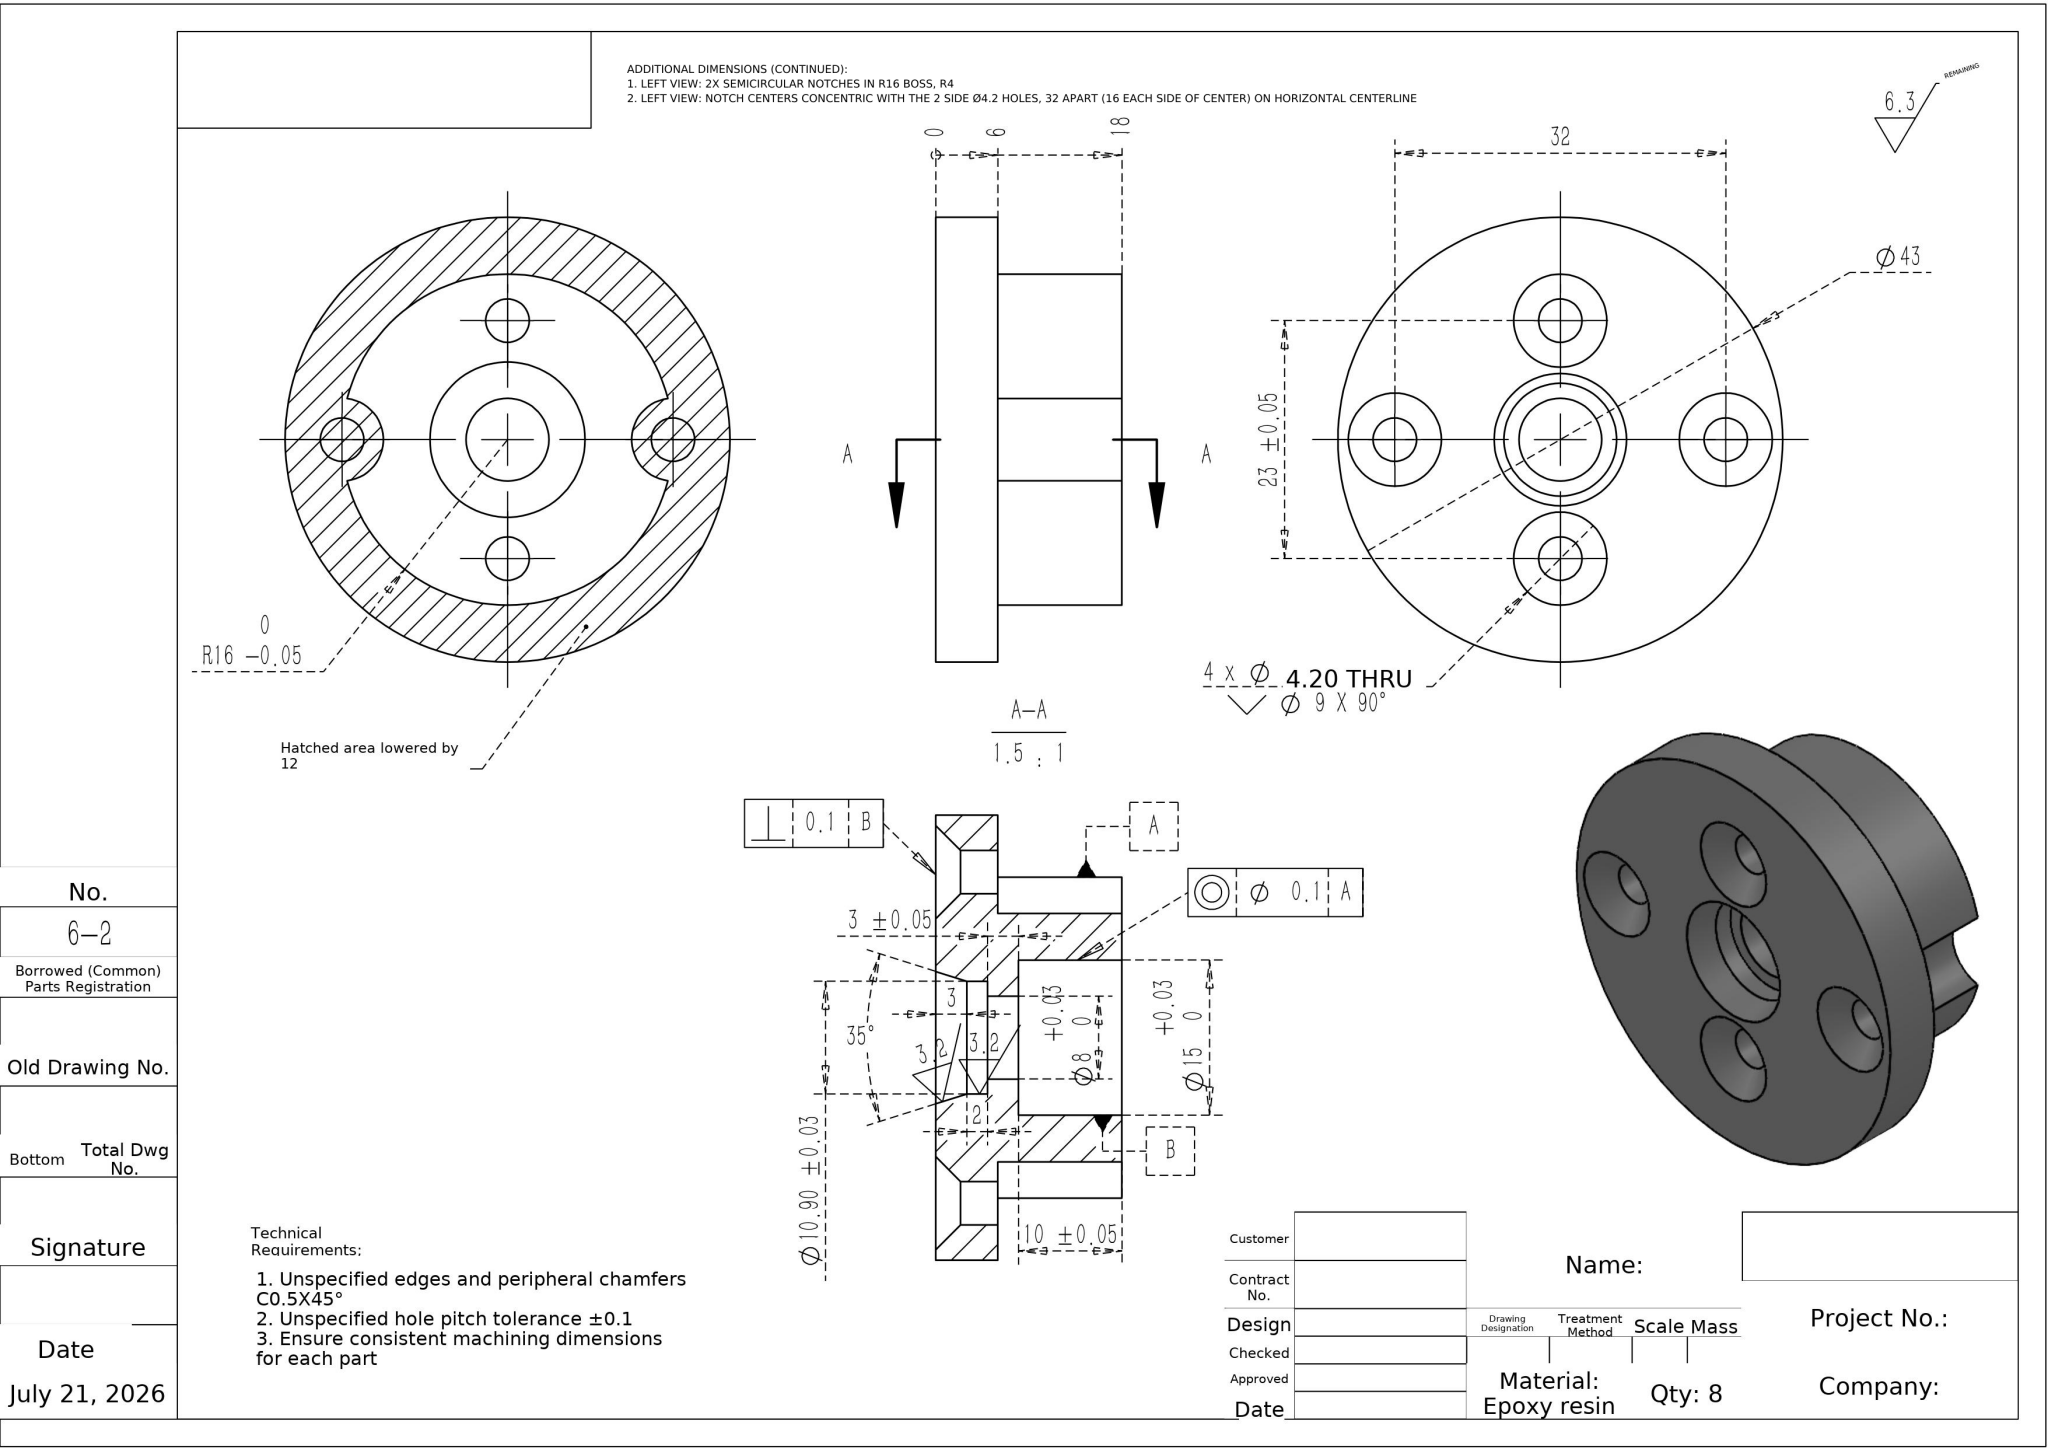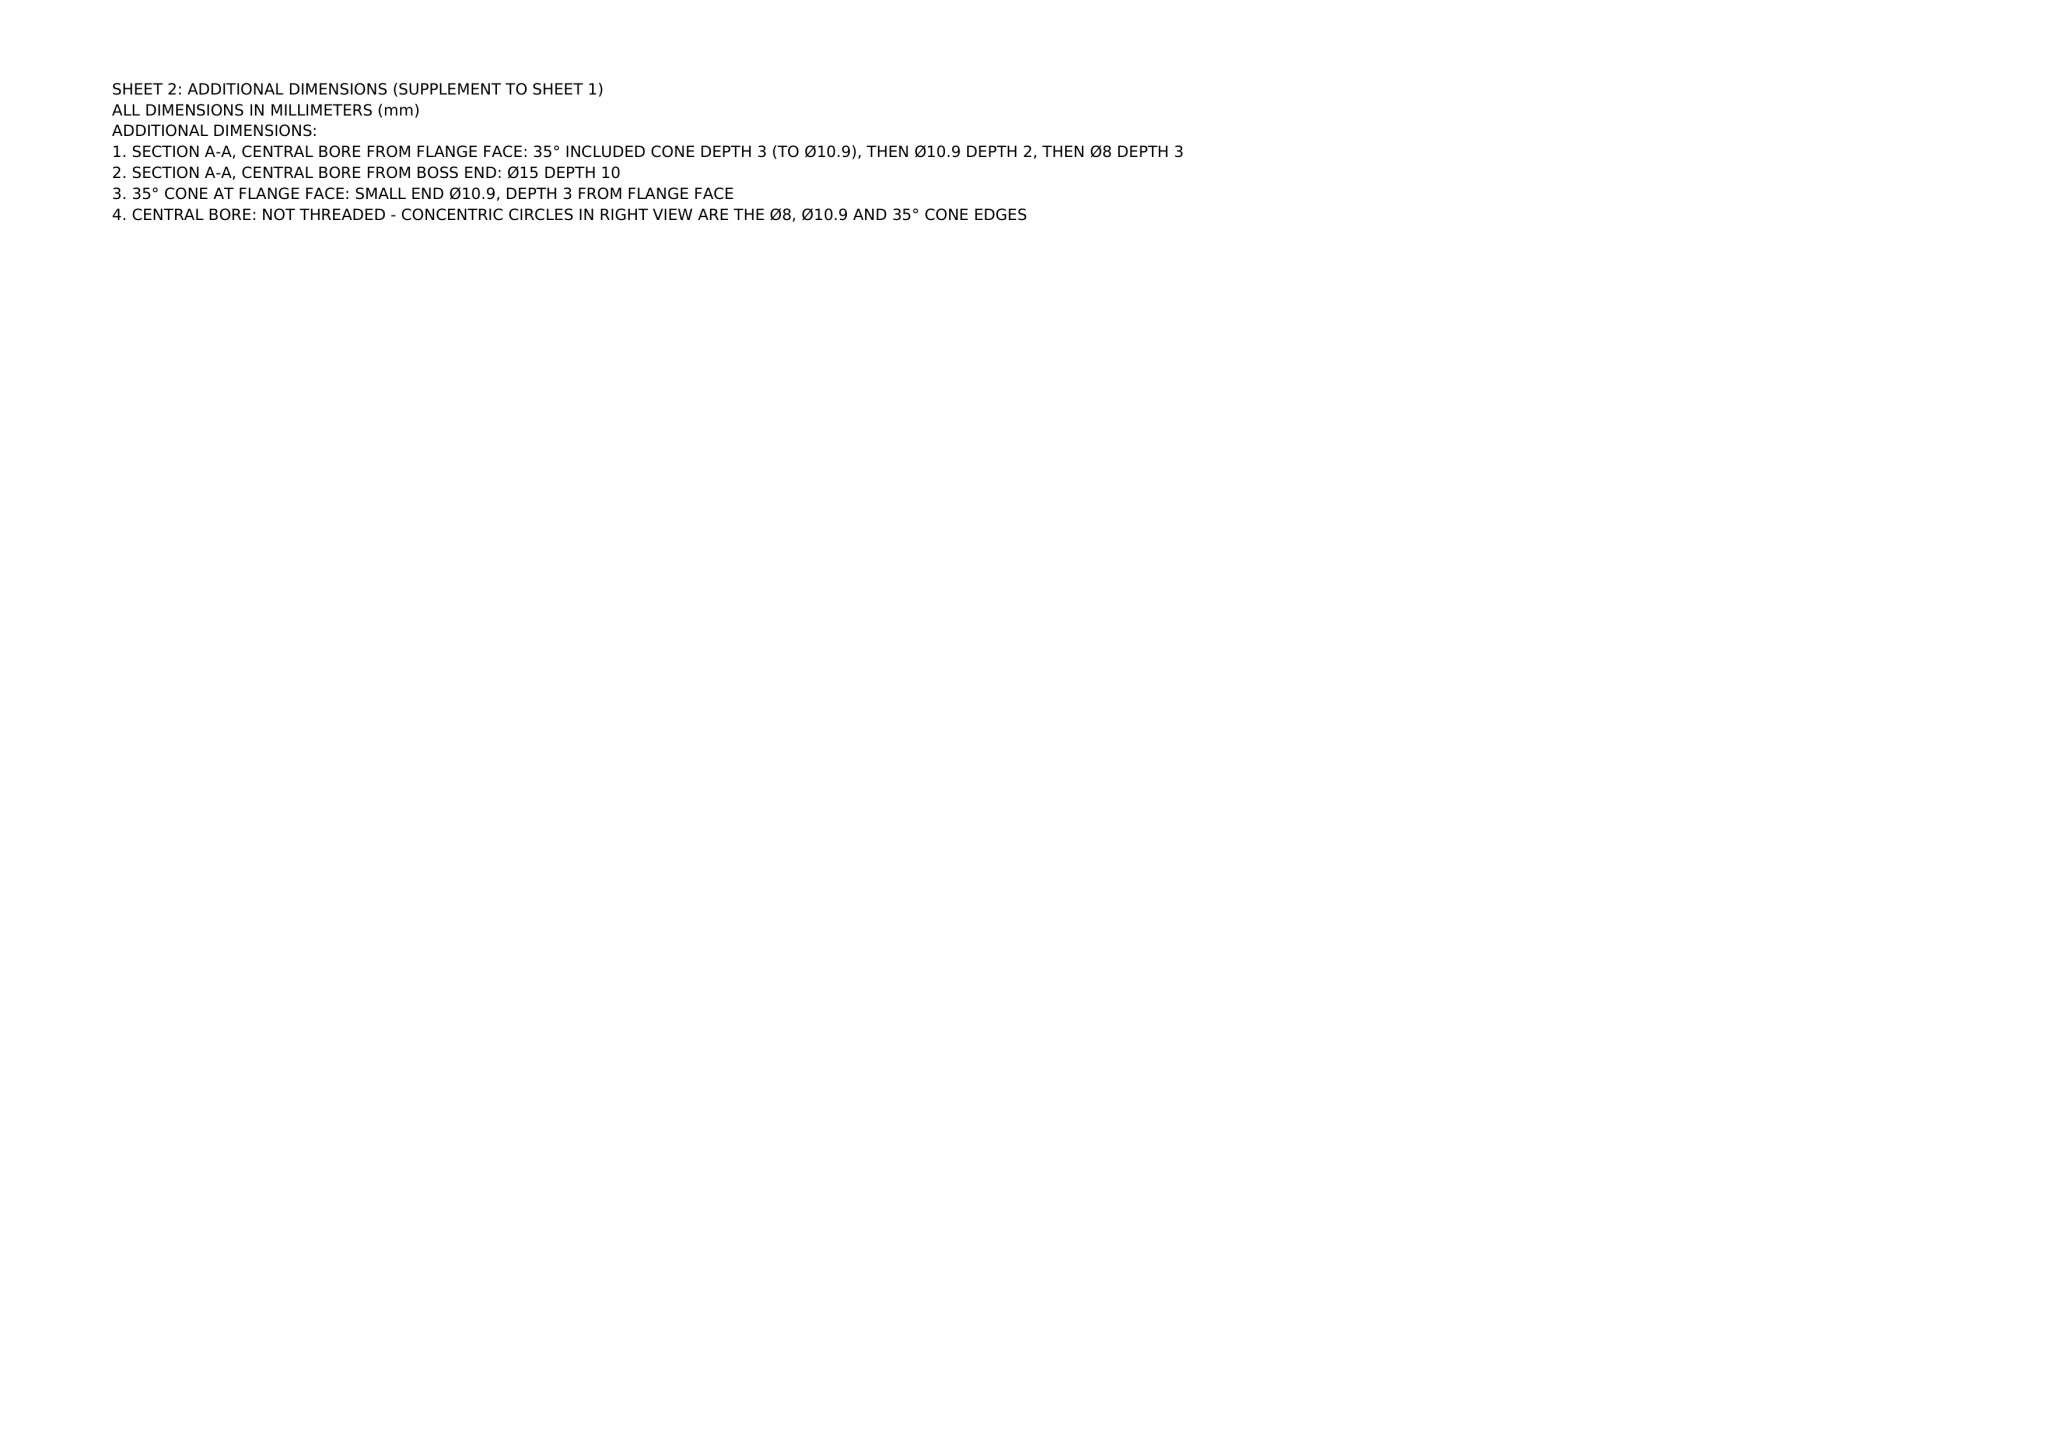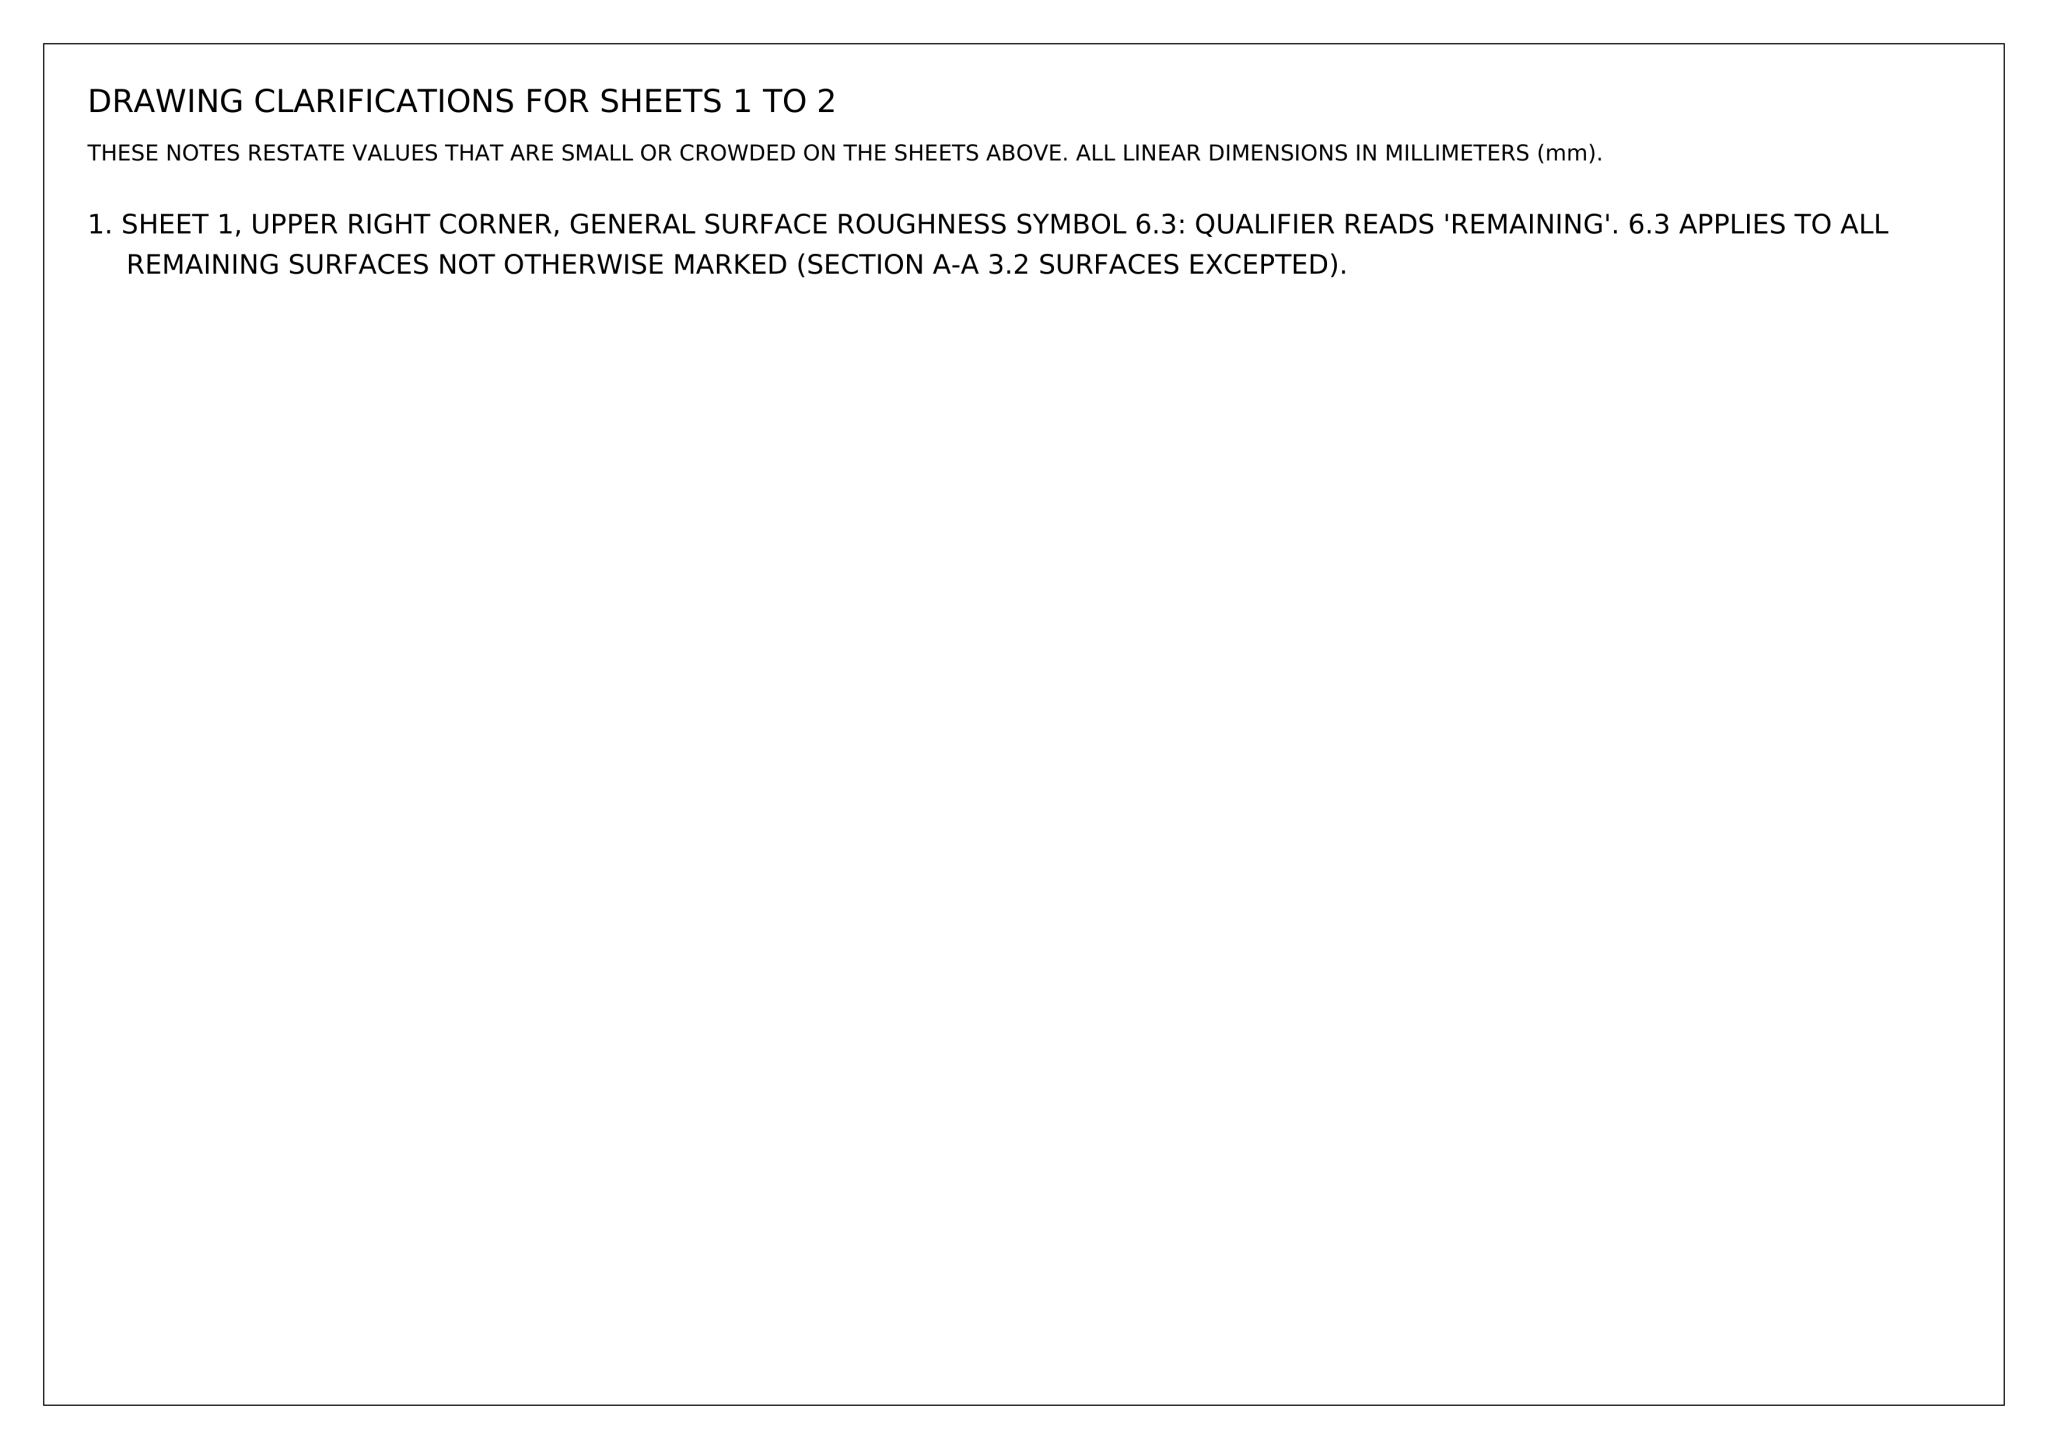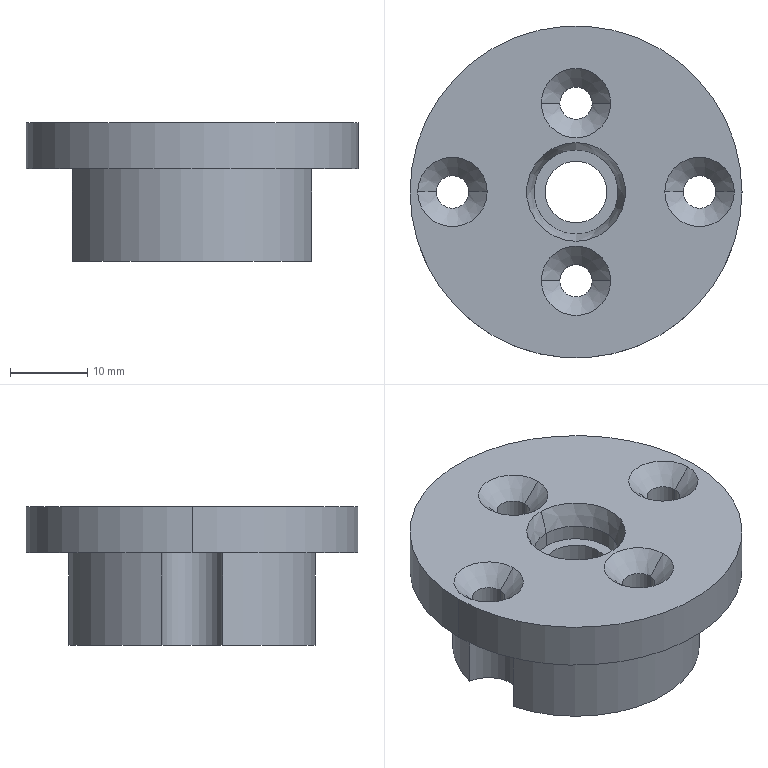Part | NX | mm | 1 solid | 36 faces | box 43 x 43 x 18 mm | volume 14482 mm3 | cylinder 21 | cone 10 | plane 5 | commonest cylinder face diameters 4.2 x8 8 x5 15 x2 10.9 x2 43 x2 32 x2